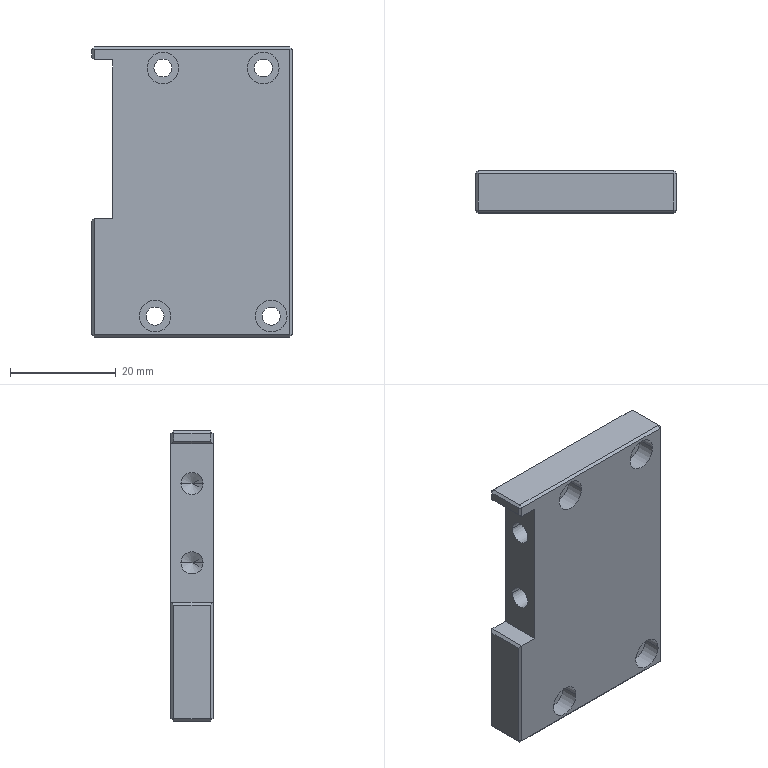Component | SolidWorks | XM-WST05-2002-1 | 1 solid | 62 faces | box 38 x 8 x 55 mm | volume 14754 mm3 | plane 38 | cylinder 20 | cone 4 | commonest cylinder face diameters 6 x8 3.4 x8 4.2 x4
build123d program:
from build123d import *

# Parameters (mm, degrees)
SKETCH1_W                                            = 38
SKETCH1_H                                            = 55
BOSS_EXTRUDE1_DEPTH                                  = 8
SKETCH2_W                                            = 8
SKETCH2_H                                            = 30
CUT_EXTRUDE1_DEPTH                                   = 35.369
HOLE_SIZE_ACCORDING_TO_HEXAGON_SOCKET_HE_D           = 3.4
HOLE_SIZE_ACCORDING_TO_HEXAGON_SOCKET_HE_CBORE_D     = 6
HOLE_SIZE_ACCORDING_TO_HEXAGON_SOCKET_HE_CBORE_DEPTH = 3.4
M5_TAPPED_HOLE1_D                                    = 4.2
M5_TAPPED_HOLE1_DEPTH                                = 14.4
M5_TAPPED_HOLE1_TIP                                  = 1.262
CHAMFER1_SIZE                                        = 0.5


with BuildPart() as part:
    # Sketch1 → Boss-Extrude1 (new body)
    with BuildSketch(Plane.XY):
        Rectangle(SKETCH1_W, SKETCH1_H)
    extrude(amount=BOSS_EXTRUDE1_DEPTH)

    # Sketch2 → Cut-Extrude1 (cut, through all)
    with BuildSketch(Plane.XY.offset(8)):
        with Locations((-19, -10)):
            Rectangle(SKETCH2_W, SKETCH2_H)
    extrude(amount=-CUT_EXTRUDE1_DEPTH, mode=Mode.SUBTRACT)

    # Hole Size according to Hexagon Socket He (through all)
    with Locations(Plane(origin=(0, 0, 0), x_dir=(-1, 0, 0), z_dir=(0, 0, -1))):
        with Locations((-15, 23.5), (7, 23.5), (-13.5, -23.476), (5.5, -23.476)):
            CounterBoreHole(HOLE_SIZE_ACCORDING_TO_HEXAGON_SOCKET_HE_D / 2, HOLE_SIZE_ACCORDING_TO_HEXAGON_SOCKET_HE_CBORE_D / 2, HOLE_SIZE_ACCORDING_TO_HEXAGON_SOCKET_HE_CBORE_DEPTH)

    # M5 Tapped Hole1
    with Locations(Plane.ZY.offset(15)):
        with Locations((4, -17.5), (4, -2.5)):
            Hole(M5_TAPPED_HOLE1_D / 2, depth=M5_TAPPED_HOLE1_DEPTH)
            with Locations((0, 0, -(M5_TAPPED_HOLE1_DEPTH + M5_TAPPED_HOLE1_TIP / 2))):  # 118° drill point
                Cone(0, M5_TAPPED_HOLE1_D / 2, M5_TAPPED_HOLE1_TIP, mode=Mode.SUBTRACT)

    # Chamfer1
    chamfer1_edges = [part.edges().sort_by_distance(p)[0] for p in [
        (19, 0, 8),
        (0, 27.5, 8),
        (-19, -26.25, 0),
        (-19, -26.25, 8),
        (-19, -25, 4),
        (-19, 5, 4),
        (-19, 16.25, 8),
        (0, 27.5, 0),
        (19, 0, 0),
        (0, -27.5, 0),
        (-19, 16.25, 0),
        (0, -27.5, 8),
        (-19, 27.5, 4),
        (19, 27.5, 4),
        (19, -27.5, 4),
        (-19, -27.5, 4),
    ]]
    chamfer(chamfer1_edges, length=CHAMFER1_SIZE)


solid = part.part

# Placed as in the assembly
solid = solid.moved(Location((-150.071, 196.819, 445.899), (-90, 0, 0)))